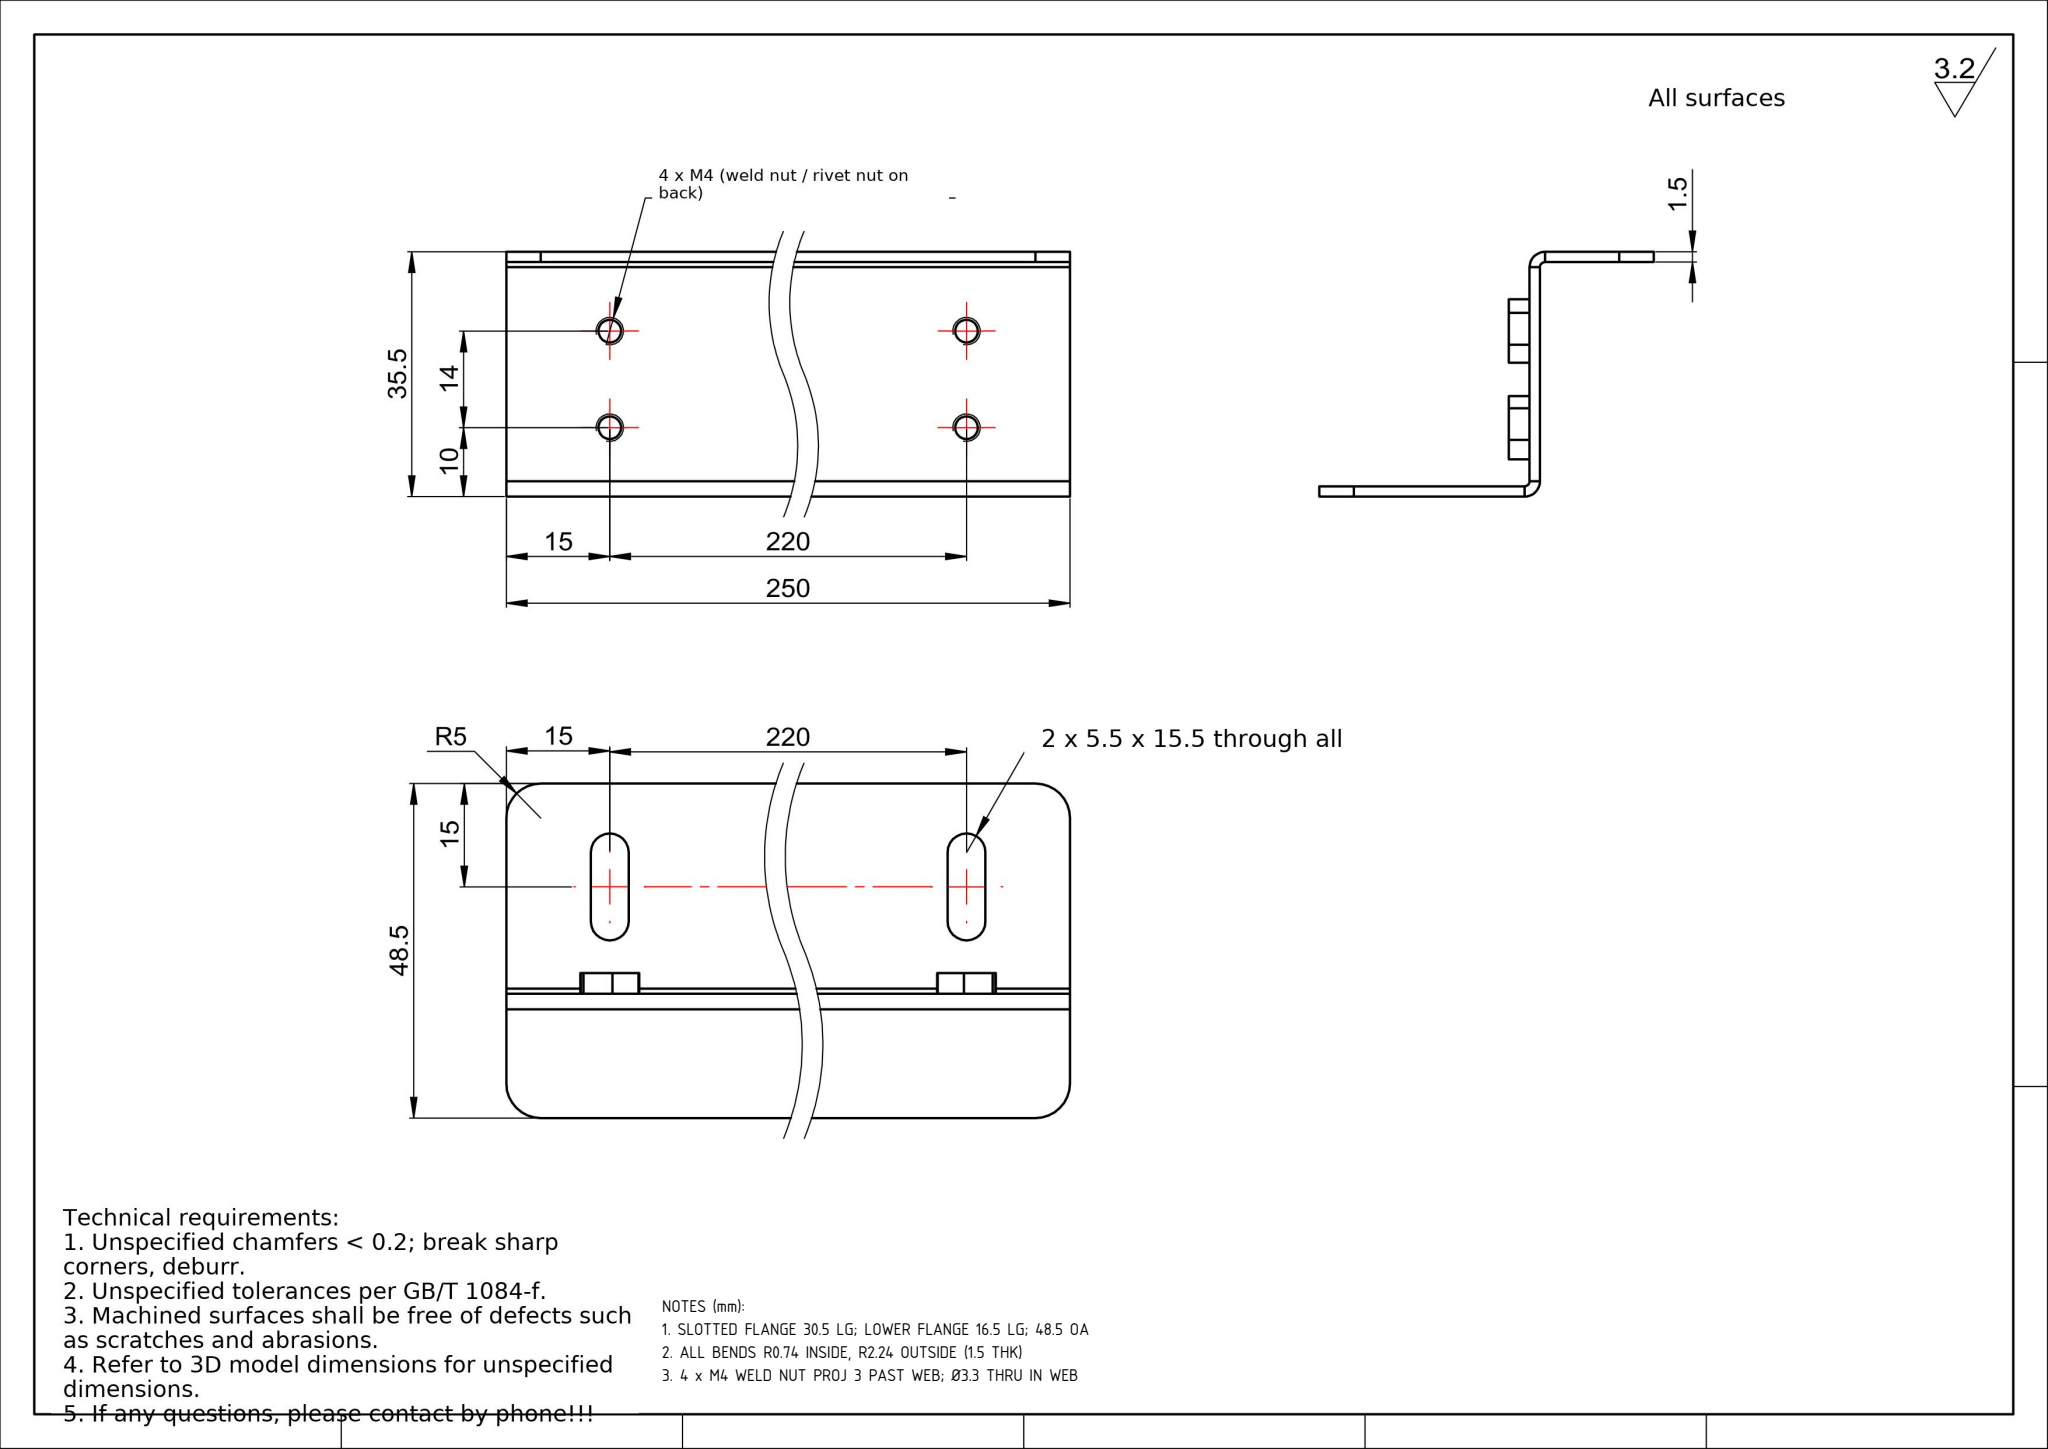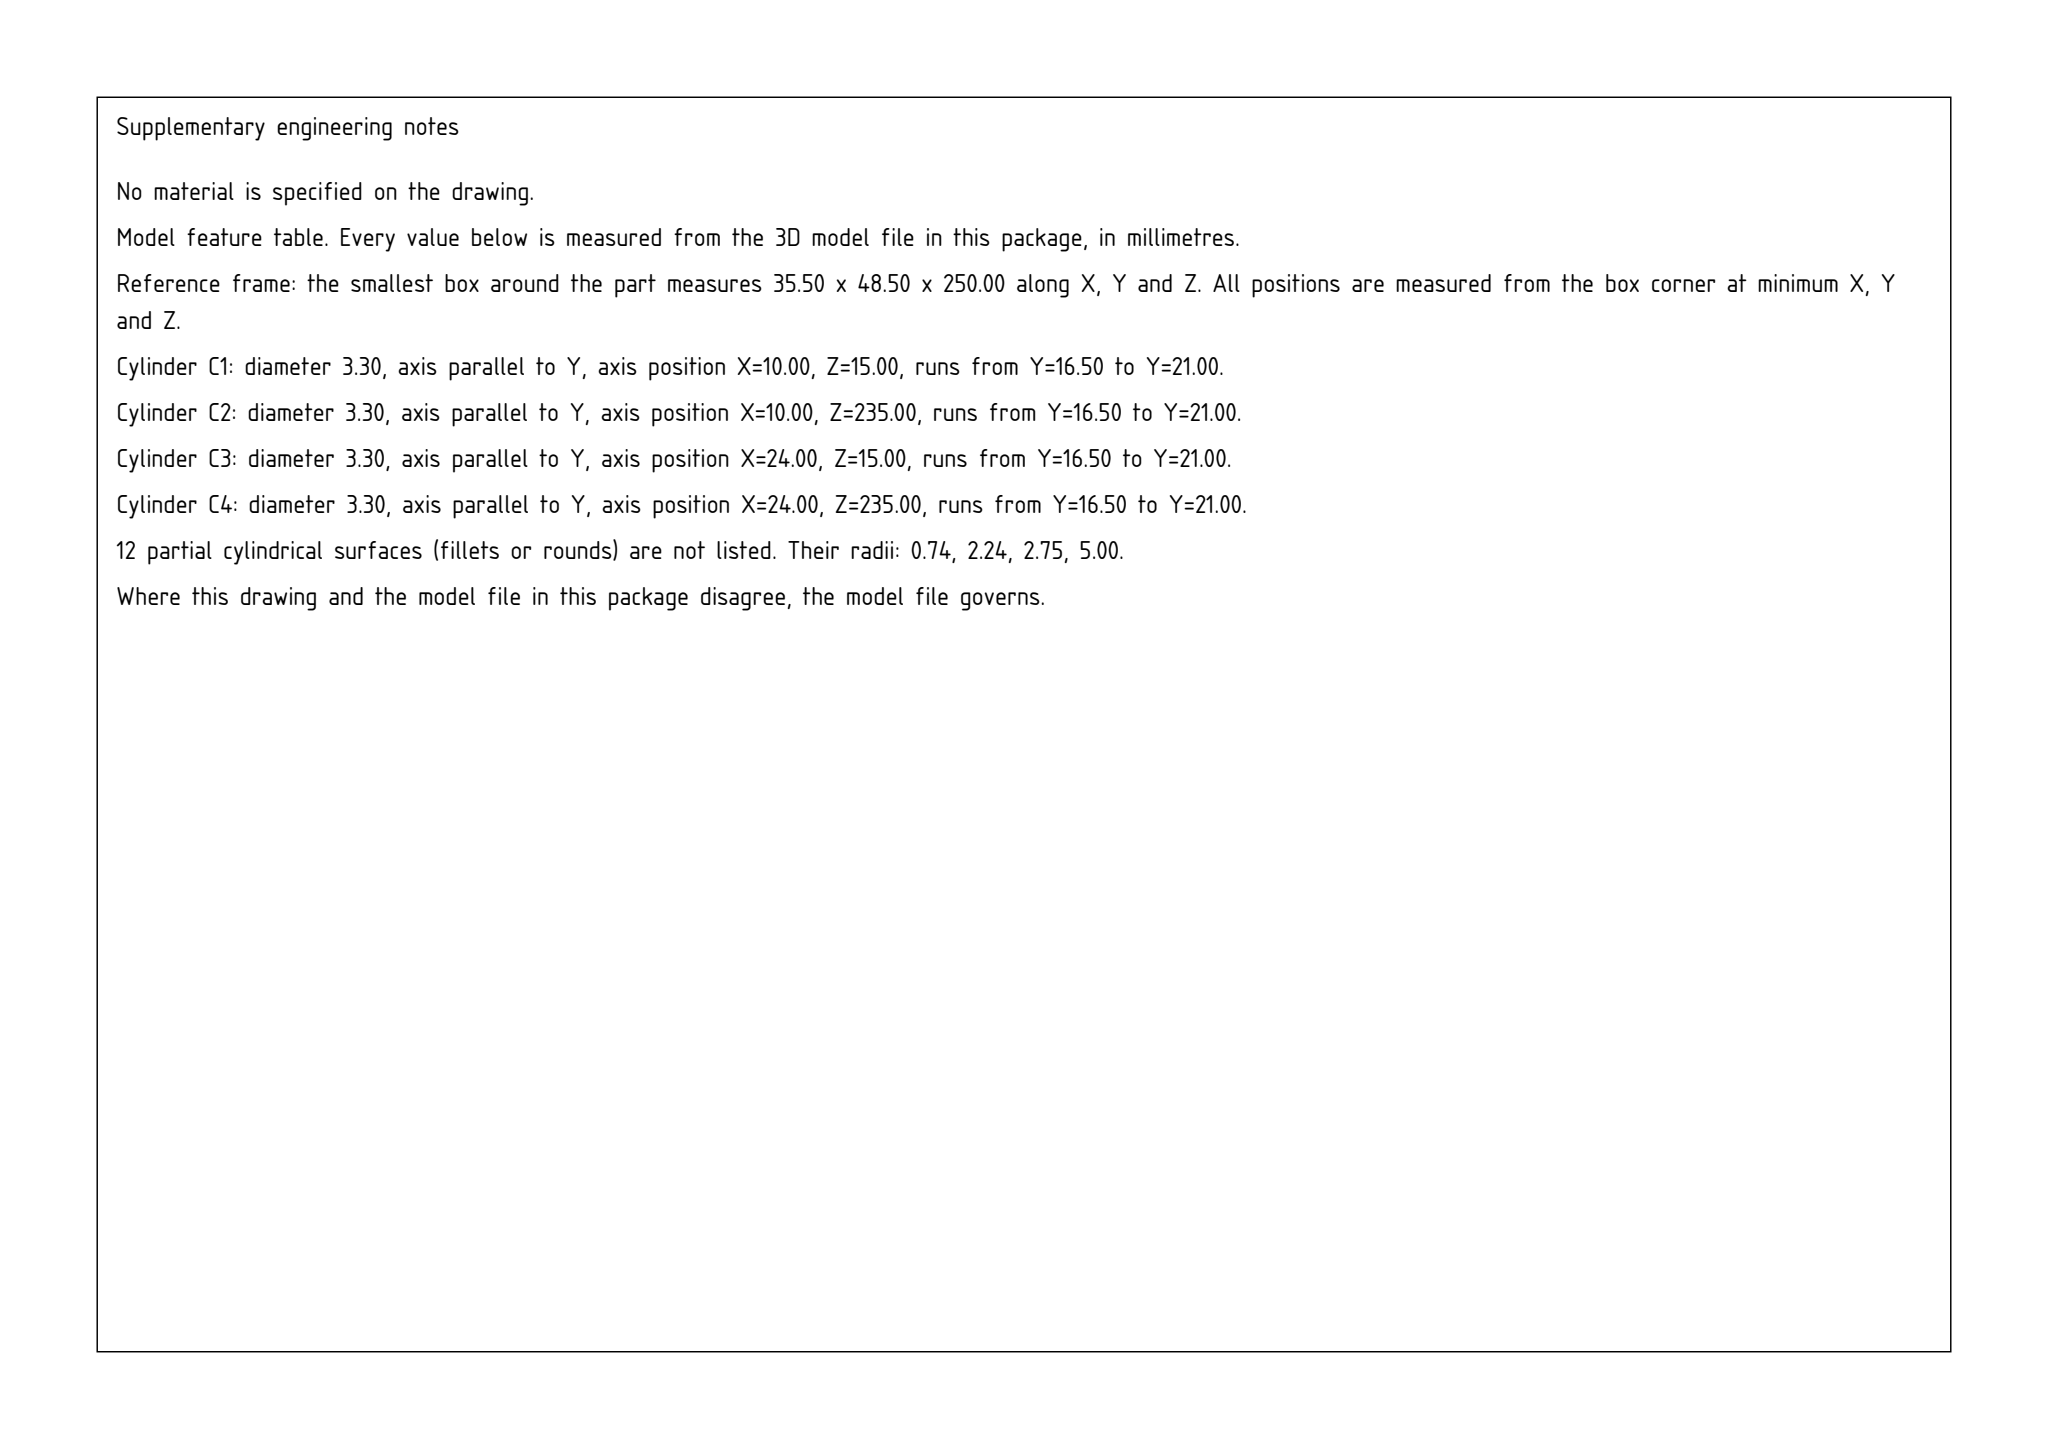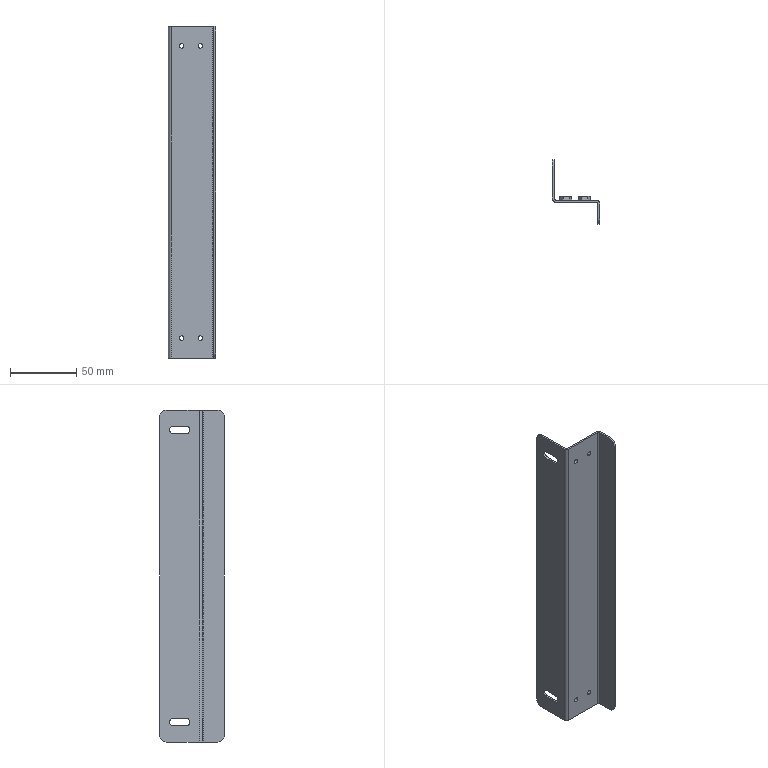Part | SolidWorks | mm | 1 solid | 70 faces | box 35.5 x 48.5 x 250 mm | volume 30702 mm3 | plane 50 | cylinder 20 | commonest cylinder face diameters 3.3 x8 5.5 x4 10 x4 4.473 x2 1.473 x2
Drawing notes:
SLOTTED FLANGE 30.5 LG; LOWER FLANGE 16.5 LG; 48.5 OA | from the solid: y-planes 0/16.5/18/48.5 with 1.5 web: 16.5 + 1.5 + 30.5 = 48.5 bbox Y
ALL BENDS R0.74 INSIDE, R2.24 OUTSIDE (1.5 THK) | from the solid: Dia 1.473 (R0.74) and 4.473 (R2.24) z-axis cyls at (2.24,18.74) & (33.26,15.76), L=250
4 x M4 WELD NUT PROJ 3 PAST WEB; Ø3.3 THRU IN WEB | from the solid: Ø3.3 y-axis holes L=4.5 from y16.5 to y21 (4x plane y=21) at z=15 & 235